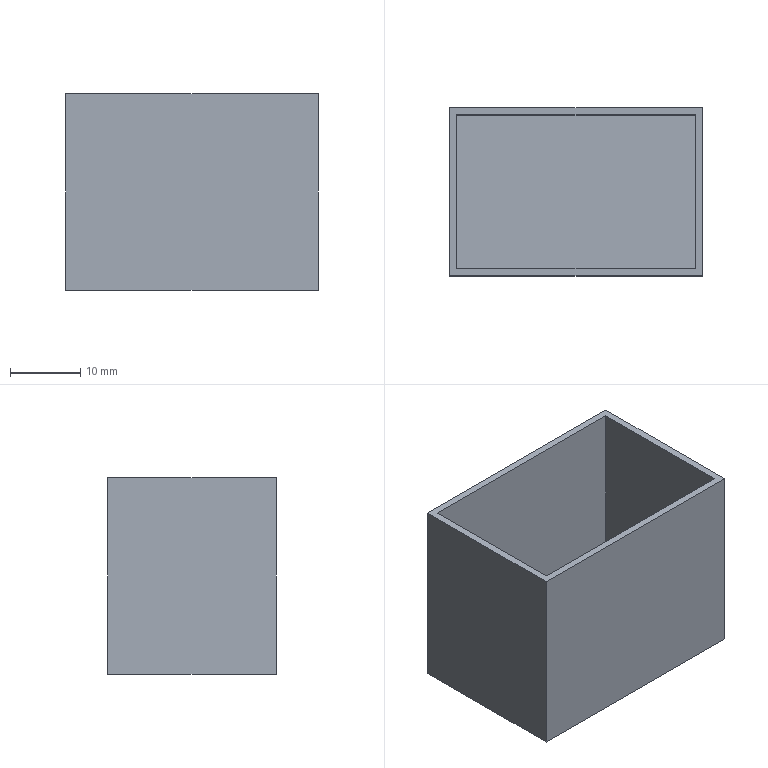Component | NX | MATERIAL_COLLECTION_BOX | 1 solid | 11 faces | box 36 x 24 x 28 mm | volume 3996 mm3 | plane 11
STEP:
#1=CARTESIAN_POINT('',(0.,0.,0.));
#2=DIRECTION('',(0.,0.,1.));
#3=DIRECTION('',(1.,0.,0.));
#4=AXIS2_PLACEMENT_3D('',#1,#2,#3);
#5=CARTESIAN_POINT('',(-110.,4.498,6.));
#6=VERTEX_POINT('',#5);
#7=CARTESIAN_POINT('',(-146.,4.498,6.));
#8=VERTEX_POINT('',#7);
#9=CARTESIAN_POINT('',(-128.,4.498,6.));
#10=DIRECTION('',(-1.,0.,0.));
#11=VECTOR('',#10,1.);
#12=LINE('',#9,#11);
#13=CARTESIAN_POINT('',(-128.,16.498,6.));
#14=DIRECTION('',(0.,0.,1.));
#15=DIRECTION('',(1.,0.,0.));
#16=AXIS2_PLACEMENT_3D('',#13,#14,#15);
#17=PLANE('',#16);
#18=CARTESIAN_POINT('',(0.,-12.));
#19=DIRECTION('',(-1.,0.));
#20=VECTOR('',#19,1.);
#21=LINE('',#18,#20);
#22=(GEOMETRIC_REPRESENTATION_CONTEXT(2)PARAMETRIC_REPRESENTATION_CONTEXT()REPRESENTATION_CONTEXT('',''));
#23=DEFINITIONAL_REPRESENTATION('',(#21),#22);
#24=PCURVE('',#17,#23);
#25=CARTESIAN_POINT('',(-128.,4.498,-22.));
#26=DIRECTION('',(0.,-1.,0.));
#27=DIRECTION('',(0.,0.,-1.));
#28=AXIS2_PLACEMENT_3D('',#25,#26,#27);
#29=PLANE('',#28);
#30=CARTESIAN_POINT('',(-28.,0.));
#31=DIRECTION('',(0.,-1.));
#32=VECTOR('',#31,1.);
#33=LINE('',#30,#32);
#34=(GEOMETRIC_REPRESENTATION_CONTEXT(2)PARAMETRIC_REPRESENTATION_CONTEXT()REPRESENTATION_CONTEXT('',''));
#35=DEFINITIONAL_REPRESENTATION('',(#33),#34);
#36=PCURVE('',#29,#35);
#37=SURFACE_CURVE('',#12,(#24,#36),.PCURVE_S1.);
#38=EDGE_CURVE('',#6,#8,#37,.T.);
#39=ORIENTED_EDGE('',*,*,#38,.F.);
#40=CARTESIAN_POINT('',(-110.,28.498,6.));
#41=VERTEX_POINT('',#40);
#42=CARTESIAN_POINT('',(-110.,16.498,6.));
#43=DIRECTION('',(0.,-1.,0.));
#44=VECTOR('',#43,1.);
#45=LINE('',#42,#44);
#46=CARTESIAN_POINT('',(18.,0.));
#47=DIRECTION('',(0.,-1.));
#48=VECTOR('',#47,1.);
#49=LINE('',#46,#48);
#50=(GEOMETRIC_REPRESENTATION_CONTEXT(2)PARAMETRIC_REPRESENTATION_CONTEXT()REPRESENTATION_CONTEXT('',''));
#51=DEFINITIONAL_REPRESENTATION('',(#49),#50);
#52=PCURVE('',#17,#51);
#53=CARTESIAN_POINT('',(-110.,16.498,-22.));
#54=DIRECTION('',(1.,0.,0.));
#55=DIRECTION('',(0.,0.,-1.));
#56=AXIS2_PLACEMENT_3D('',#53,#54,#55);
#57=PLANE('',#56);
#58=CARTESIAN_POINT('',(-28.,0.));
#59=DIRECTION('',(0.,-1.));
#60=VECTOR('',#59,1.);
#61=LINE('',#58,#60);
#62=(GEOMETRIC_REPRESENTATION_CONTEXT(2)PARAMETRIC_REPRESENTATION_CONTEXT()REPRESENTATION_CONTEXT('',''));
#63=DEFINITIONAL_REPRESENTATION('',(#61),#62);
#64=PCURVE('',#57,#63);
#65=SURFACE_CURVE('',#45,(#52,#64),.PCURVE_S1.);
#66=EDGE_CURVE('',#41,#6,#65,.T.);
#67=ORIENTED_EDGE('',*,*,#66,.F.);
#68=CARTESIAN_POINT('',(-146.,28.498,6.));
#69=VERTEX_POINT('',#68);
#70=CARTESIAN_POINT('',(-128.,28.498,6.));
#71=DIRECTION('',(1.,0.,0.));
#72=VECTOR('',#71,1.);
#73=LINE('',#70,#72);
#74=CARTESIAN_POINT('',(0.,12.));
#75=DIRECTION('',(1.,0.));
#76=VECTOR('',#75,1.);
#77=LINE('',#74,#76);
#78=(GEOMETRIC_REPRESENTATION_CONTEXT(2)PARAMETRIC_REPRESENTATION_CONTEXT()REPRESENTATION_CONTEXT('',''));
#79=DEFINITIONAL_REPRESENTATION('',(#77),#78);
#80=PCURVE('',#17,#79);
#81=CARTESIAN_POINT('',(-128.,28.498,-22.));
#82=DIRECTION('',(0.,1.,0.));
#83=DIRECTION('',(0.,0.,1.));
#84=AXIS2_PLACEMENT_3D('',#81,#82,#83);
#85=PLANE('',#84);
#86=CARTESIAN_POINT('',(28.,0.));
#87=DIRECTION('',(0.,1.));
#88=VECTOR('',#87,1.);
#89=LINE('',#86,#88);
#90=(GEOMETRIC_REPRESENTATION_CONTEXT(2)PARAMETRIC_REPRESENTATION_CONTEXT()REPRESENTATION_CONTEXT('',''));
#91=DEFINITIONAL_REPRESENTATION('',(#89),#90);
#92=PCURVE('',#85,#91);
#93=SURFACE_CURVE('',#73,(#80,#92),.PCURVE_S1.);
#94=EDGE_CURVE('',#69,#41,#93,.T.);
#95=ORIENTED_EDGE('',*,*,#94,.F.);
#96=CARTESIAN_POINT('',(-146.,16.498,6.));
#97=DIRECTION('',(0.,1.,0.));
#98=VECTOR('',#97,1.);
#99=LINE('',#96,#98);
#100=CARTESIAN_POINT('',(-18.,0.));
#101=DIRECTION('',(0.,1.));
#102=VECTOR('',#101,1.);
#103=LINE('',#100,#102);
#104=(GEOMETRIC_REPRESENTATION_CONTEXT(2)PARAMETRIC_REPRESENTATION_CONTEXT()REPRESENTATION_CONTEXT('',''));
#105=DEFINITIONAL_REPRESENTATION('',(#103),#104);
#106=PCURVE('',#17,#105);
#107=CARTESIAN_POINT('',(-146.,16.498,-22.));
#108=DIRECTION('',(-1.,0.,0.));
#109=DIRECTION('',(0.,0.,1.));
#110=AXIS2_PLACEMENT_3D('',#107,#108,#109);
#111=PLANE('',#110);
#112=CARTESIAN_POINT('',(28.,0.));
#113=DIRECTION('',(0.,1.));
#114=VECTOR('',#113,1.);
#115=LINE('',#112,#114);
#116=(GEOMETRIC_REPRESENTATION_CONTEXT(2)PARAMETRIC_REPRESENTATION_CONTEXT()REPRESENTATION_CONTEXT('',''));
#117=DEFINITIONAL_REPRESENTATION('',(#115),#116);
#118=PCURVE('',#111,#117);
#119=SURFACE_CURVE('',#99,(#106,#118),.PCURVE_S1.);
#120=EDGE_CURVE('',#8,#69,#119,.T.);
#121=ORIENTED_EDGE('',*,*,#120,.F.);
#122=EDGE_LOOP('',(#39,#67,#95,#121));
#123=FACE_BOUND('',#122,.T.);
#124=CARTESIAN_POINT('',(-111.,27.498,6.));
#125=VERTEX_POINT('',#124);
#126=CARTESIAN_POINT('',(-111.,5.498,6.));
#127=VERTEX_POINT('',#126);
#128=CARTESIAN_POINT('',(-111.,16.498,6.));
#129=DIRECTION('',(0.,-1.,0.));
#130=VECTOR('',#129,1.);
#131=LINE('',#128,#130);
#132=CARTESIAN_POINT('',(17.,0.));
#133=DIRECTION('',(0.,-1.));
#134=VECTOR('',#133,1.);
#135=LINE('',#132,#134);
#136=(GEOMETRIC_REPRESENTATION_CONTEXT(2)PARAMETRIC_REPRESENTATION_CONTEXT()REPRESENTATION_CONTEXT('',''));
#137=DEFINITIONAL_REPRESENTATION('',(#135),#136);
#138=PCURVE('',#17,#137);
#139=CARTESIAN_POINT('',(-111.,16.498,-22.));
#140=DIRECTION('',(1.,0.,0.));
#141=DIRECTION('',(0.,0.,-1.));
#142=AXIS2_PLACEMENT_3D('',#139,#140,#141);
#143=PLANE('',#142);
#144=CARTESIAN_POINT('',(-28.,0.));
#145=DIRECTION('',(0.,-1.));
#146=VECTOR('',#145,1.);
#147=LINE('',#144,#146);
#148=(GEOMETRIC_REPRESENTATION_CONTEXT(2)PARAMETRIC_REPRESENTATION_CONTEXT()REPRESENTATION_CONTEXT('',''));
#149=DEFINITIONAL_REPRESENTATION('',(#147),#148);
#150=PCURVE('',#143,#149);
#151=SURFACE_CURVE('',#131,(#138,#150),.PCURVE_S1.);
#152=EDGE_CURVE('',#125,#127,#151,.T.);
#153=ORIENTED_EDGE('',*,*,#152,.T.);
#154=CARTESIAN_POINT('',(-145.,5.498,6.));
#155=VERTEX_POINT('',#154);
#156=CARTESIAN_POINT('',(-128.,5.498,6.));
#157=DIRECTION('',(-1.,0.,0.));
#158=VECTOR('',#157,1.);
#159=LINE('',#156,#158);
#160=CARTESIAN_POINT('',(0.,-11.));
#161=DIRECTION('',(-1.,0.));
#162=VECTOR('',#161,1.);
#163=LINE('',#160,#162);
#164=(GEOMETRIC_REPRESENTATION_CONTEXT(2)PARAMETRIC_REPRESENTATION_CONTEXT()REPRESENTATION_CONTEXT('',''));
#165=DEFINITIONAL_REPRESENTATION('',(#163),#164);
#166=PCURVE('',#17,#165);
#167=CARTESIAN_POINT('',(-128.,5.498,-22.));
#168=DIRECTION('',(0.,-1.,0.));
#169=DIRECTION('',(0.,0.,-1.));
#170=AXIS2_PLACEMENT_3D('',#167,#168,#169);
#171=PLANE('',#170);
#172=CARTESIAN_POINT('',(-28.,0.));
#173=DIRECTION('',(0.,-1.));
#174=VECTOR('',#173,1.);
#175=LINE('',#172,#174);
#176=(GEOMETRIC_REPRESENTATION_CONTEXT(2)PARAMETRIC_REPRESENTATION_CONTEXT()REPRESENTATION_CONTEXT('',''));
#177=DEFINITIONAL_REPRESENTATION('',(#175),#176);
#178=PCURVE('',#171,#177);
#179=SURFACE_CURVE('',#159,(#166,#178),.PCURVE_S1.);
#180=EDGE_CURVE('',#127,#155,#179,.T.);
#181=ORIENTED_EDGE('',*,*,#180,.T.);
#182=CARTESIAN_POINT('',(-145.,27.498,6.));
#183=VERTEX_POINT('',#182);
#184=CARTESIAN_POINT('',(-145.,16.498,6.));
#185=DIRECTION('',(0.,1.,0.));
#186=VECTOR('',#185,1.);
#187=LINE('',#184,#186);
#188=CARTESIAN_POINT('',(-17.,0.));
#189=DIRECTION('',(0.,1.));
#190=VECTOR('',#189,1.);
#191=LINE('',#188,#190);
#192=(GEOMETRIC_REPRESENTATION_CONTEXT(2)PARAMETRIC_REPRESENTATION_CONTEXT()REPRESENTATION_CONTEXT('',''));
#193=DEFINITIONAL_REPRESENTATION('',(#191),#192);
#194=PCURVE('',#17,#193);
#195=CARTESIAN_POINT('',(-145.,16.498,-22.));
#196=DIRECTION('',(-1.,0.,0.));
#197=DIRECTION('',(0.,0.,1.));
#198=AXIS2_PLACEMENT_3D('',#195,#196,#197);
#199=PLANE('',#198);
#200=CARTESIAN_POINT('',(28.,0.));
#201=DIRECTION('',(0.,1.));
#202=VECTOR('',#201,1.);
#203=LINE('',#200,#202);
#204=(GEOMETRIC_REPRESENTATION_CONTEXT(2)PARAMETRIC_REPRESENTATION_CONTEXT()REPRESENTATION_CONTEXT('',''));
#205=DEFINITIONAL_REPRESENTATION('',(#203),#204);
#206=PCURVE('',#199,#205);
#207=SURFACE_CURVE('',#187,(#194,#206),.PCURVE_S1.);
#208=EDGE_CURVE('',#155,#183,#207,.T.);
#209=ORIENTED_EDGE('',*,*,#208,.T.);
#210=CARTESIAN_POINT('',(-128.,27.498,6.));
#211=DIRECTION('',(1.,0.,0.));
#212=VECTOR('',#211,1.);
#213=LINE('',#210,#212);
#214=CARTESIAN_POINT('',(0.,11.));
#215=DIRECTION('',(1.,0.));
#216=VECTOR('',#215,1.);
#217=LINE('',#214,#216);
#218=(GEOMETRIC_REPRESENTATION_CONTEXT(2)PARAMETRIC_REPRESENTATION_CONTEXT()REPRESENTATION_CONTEXT('',''));
#219=DEFINITIONAL_REPRESENTATION('',(#217),#218);
#220=PCURVE('',#17,#219);
#221=CARTESIAN_POINT('',(-128.,27.498,-22.));
#222=DIRECTION('',(0.,1.,0.));
#223=DIRECTION('',(0.,0.,1.));
#224=AXIS2_PLACEMENT_3D('',#221,#222,#223);
#225=PLANE('',#224);
#226=CARTESIAN_POINT('',(28.,0.));
#227=DIRECTION('',(0.,1.));
#228=VECTOR('',#227,1.);
#229=LINE('',#226,#228);
#230=(GEOMETRIC_REPRESENTATION_CONTEXT(2)PARAMETRIC_REPRESENTATION_CONTEXT()REPRESENTATION_CONTEXT('',''));
#231=DEFINITIONAL_REPRESENTATION('',(#229),#230);
#232=PCURVE('',#225,#231);
#233=SURFACE_CURVE('',#213,(#220,#232),.PCURVE_S1.);
#234=EDGE_CURVE('',#183,#125,#233,.T.);
#235=ORIENTED_EDGE('',*,*,#234,.T.);
#236=EDGE_LOOP('',(#153,#181,#209,#235));
#237=FACE_BOUND('',#236,.T.);
#238=ADVANCED_FACE('',(#123,#237),#17,.T.);
#239=CARTESIAN_POINT('',(-110.,4.498,-22.));
#240=VERTEX_POINT('',#239);
#241=CARTESIAN_POINT('',(-110.,4.498,-22.));
#242=DIRECTION('',(0.,0.,1.));
#243=VECTOR('',#242,1.);
#244=LINE('',#241,#243);
#245=CARTESIAN_POINT('',(0.,18.));
#246=DIRECTION('',(-1.,0.));
#247=VECTOR('',#246,1.);
#248=LINE('',#245,#247);
#249=(GEOMETRIC_REPRESENTATION_CONTEXT(2)PARAMETRIC_REPRESENTATION_CONTEXT()REPRESENTATION_CONTEXT('',''));
#250=DEFINITIONAL_REPRESENTATION('',(#248),#249);
#251=PCURVE('',#29,#250);
#252=CARTESIAN_POINT('',(0.,-12.));
#253=DIRECTION('',(-1.,0.));
#254=VECTOR('',#253,1.);
#255=LINE('',#252,#254);
#256=(GEOMETRIC_REPRESENTATION_CONTEXT(2)PARAMETRIC_REPRESENTATION_CONTEXT()REPRESENTATION_CONTEXT('',''));
#257=DEFINITIONAL_REPRESENTATION('',(#255),#256);
#258=PCURVE('',#57,#257);
#259=SURFACE_CURVE('',#244,(#251,#258),.PCURVE_S1.);
#260=EDGE_CURVE('',#240,#6,#259,.T.);
#261=ORIENTED_EDGE('',*,*,#260,.T.);
#262=ORIENTED_EDGE('',*,*,#38,.T.);
#263=CARTESIAN_POINT('',(-146.,4.498,-22.));
#264=VERTEX_POINT('',#263);
#265=CARTESIAN_POINT('',(-146.,4.498,-22.));
#266=DIRECTION('',(0.,0.,1.));
#267=VECTOR('',#266,1.);
#268=LINE('',#265,#267);
#269=CARTESIAN_POINT('',(0.,-18.));
#270=DIRECTION('',(-1.,0.));
#271=VECTOR('',#270,1.);
#272=LINE('',#269,#271);
#273=(GEOMETRIC_REPRESENTATION_CONTEXT(2)PARAMETRIC_REPRESENTATION_CONTEXT()REPRESENTATION_CONTEXT('',''));
#274=DEFINITIONAL_REPRESENTATION('',(#272),#273);
#275=PCURVE('',#29,#274);
#276=CARTESIAN_POINT('',(0.,-12.));
#277=DIRECTION('',(1.,0.));
#278=VECTOR('',#277,1.);
#279=LINE('',#276,#278);
#280=(GEOMETRIC_REPRESENTATION_CONTEXT(2)PARAMETRIC_REPRESENTATION_CONTEXT()REPRESENTATION_CONTEXT('',''));
#281=DEFINITIONAL_REPRESENTATION('',(#279),#280);
#282=PCURVE('',#111,#281);
#283=SURFACE_CURVE('',#268,(#275,#282),.PCURVE_S1.);
#284=EDGE_CURVE('',#264,#8,#283,.T.);
#285=ORIENTED_EDGE('',*,*,#284,.F.);
#286=CARTESIAN_POINT('',(-128.,4.498,-22.));
#287=DIRECTION('',(1.,0.,0.));
#288=VECTOR('',#287,1.);
#289=LINE('',#286,#288);
#290=CARTESIAN_POINT('',(0.,0.));
#291=DIRECTION('',(0.,1.));
#292=VECTOR('',#291,1.);
#293=LINE('',#290,#292);
#294=(GEOMETRIC_REPRESENTATION_CONTEXT(2)PARAMETRIC_REPRESENTATION_CONTEXT()REPRESENTATION_CONTEXT('',''));
#295=DEFINITIONAL_REPRESENTATION('',(#293),#294);
#296=PCURVE('',#29,#295);
#297=CARTESIAN_POINT('',(-128.,16.498,-22.));
#298=DIRECTION('',(0.,0.,-1.));
#299=DIRECTION('',(-1.,0.,0.));
#300=AXIS2_PLACEMENT_3D('',#297,#298,#299);
#301=PLANE('',#300);
#302=CARTESIAN_POINT('',(0.,-12.));
#303=DIRECTION('',(-1.,0.));
#304=VECTOR('',#303,1.);
#305=LINE('',#302,#304);
#306=(GEOMETRIC_REPRESENTATION_CONTEXT(2)PARAMETRIC_REPRESENTATION_CONTEXT()REPRESENTATION_CONTEXT('',''));
#307=DEFINITIONAL_REPRESENTATION('',(#305),#306);
#308=PCURVE('',#301,#307);
#309=SURFACE_CURVE('',#289,(#296,#308),.PCURVE_S1.);
#310=EDGE_CURVE('',#264,#240,#309,.T.);
#311=ORIENTED_EDGE('',*,*,#310,.T.);
#312=EDGE_LOOP('',(#261,#262,#285,#311));
#313=FACE_BOUND('',#312,.T.);
#314=ADVANCED_FACE('',(#313),#29,.T.);
#315=ORIENTED_EDGE('',*,*,#284,.T.);
#316=ORIENTED_EDGE('',*,*,#120,.T.);
#317=CARTESIAN_POINT('',(-146.,28.498,-22.));
#318=VERTEX_POINT('',#317);
#319=CARTESIAN_POINT('',(-146.,28.498,-22.));
#320=DIRECTION('',(0.,0.,1.));
#321=VECTOR('',#320,1.);
#322=LINE('',#319,#321);
#323=CARTESIAN_POINT('',(0.,12.));
#324=DIRECTION('',(1.,0.));
#325=VECTOR('',#324,1.);
#326=LINE('',#323,#325);
#327=(GEOMETRIC_REPRESENTATION_CONTEXT(2)PARAMETRIC_REPRESENTATION_CONTEXT()REPRESENTATION_CONTEXT('',''));
#328=DEFINITIONAL_REPRESENTATION('',(#326),#327);
#329=PCURVE('',#111,#328);
#330=CARTESIAN_POINT('',(0.,-18.));
#331=DIRECTION('',(1.,0.));
#332=VECTOR('',#331,1.);
#333=LINE('',#330,#332);
#334=(GEOMETRIC_REPRESENTATION_CONTEXT(2)PARAMETRIC_REPRESENTATION_CONTEXT()REPRESENTATION_CONTEXT('',''));
#335=DEFINITIONAL_REPRESENTATION('',(#333),#334);
#336=PCURVE('',#85,#335);
#337=SURFACE_CURVE('',#322,(#329,#336),.PCURVE_S1.);
#338=EDGE_CURVE('',#318,#69,#337,.T.);
#339=ORIENTED_EDGE('',*,*,#338,.F.);
#340=CARTESIAN_POINT('',(-146.,16.498,-22.));
#341=DIRECTION('',(0.,-1.,0.));
#342=VECTOR('',#341,1.);
#343=LINE('',#340,#342);
#344=CARTESIAN_POINT('',(0.,0.));
#345=DIRECTION('',(0.,-1.));
#346=VECTOR('',#345,1.);
#347=LINE('',#344,#346);
#348=(GEOMETRIC_REPRESENTATION_CONTEXT(2)PARAMETRIC_REPRESENTATION_CONTEXT()REPRESENTATION_CONTEXT('',''));
#349=DEFINITIONAL_REPRESENTATION('',(#347),#348);
#350=PCURVE('',#111,#349);
#351=CARTESIAN_POINT('',(18.,0.));
#352=DIRECTION('',(0.,-1.));
#353=VECTOR('',#352,1.);
#354=LINE('',#351,#353);
#355=(GEOMETRIC_REPRESENTATION_CONTEXT(2)PARAMETRIC_REPRESENTATION_CONTEXT()REPRESENTATION_CONTEXT('',''));
#356=DEFINITIONAL_REPRESENTATION('',(#354),#355);
#357=PCURVE('',#301,#356);
#358=SURFACE_CURVE('',#343,(#350,#357),.PCURVE_S1.);
#359=EDGE_CURVE('',#318,#264,#358,.T.);
#360=ORIENTED_EDGE('',*,*,#359,.T.);
#361=EDGE_LOOP('',(#315,#316,#339,#360));
#362=FACE_BOUND('',#361,.T.);
#363=ADVANCED_FACE('',(#362),#111,.T.);
#364=ORIENTED_EDGE('',*,*,#338,.T.);
#365=ORIENTED_EDGE('',*,*,#94,.T.);
#366=CARTESIAN_POINT('',(-110.,28.498,-22.));
#367=VERTEX_POINT('',#366);
#368=CARTESIAN_POINT('',(-110.,28.498,-22.));
#369=DIRECTION('',(0.,0.,1.));
#370=VECTOR('',#369,1.);
#371=LINE('',#368,#370);
#372=CARTESIAN_POINT('',(0.,18.));
#373=DIRECTION('',(1.,0.));
#374=VECTOR('',#373,1.);
#375=LINE('',#372,#374);
#376=(GEOMETRIC_REPRESENTATION_CONTEXT(2)PARAMETRIC_REPRESENTATION_CONTEXT()REPRESENTATION_CONTEXT('',''));
#377=DEFINITIONAL_REPRESENTATION('',(#375),#376);
#378=PCURVE('',#85,#377);
#379=CARTESIAN_POINT('',(0.,12.));
#380=DIRECTION('',(-1.,0.));
#381=VECTOR('',#380,1.);
#382=LINE('',#379,#381);
#383=(GEOMETRIC_REPRESENTATION_CONTEXT(2)PARAMETRIC_REPRESENTATION_CONTEXT()REPRESENTATION_CONTEXT('',''));
#384=DEFINITIONAL_REPRESENTATION('',(#382),#383);
#385=PCURVE('',#57,#384);
#386=SURFACE_CURVE('',#371,(#378,#385),.PCURVE_S1.);
#387=EDGE_CURVE('',#367,#41,#386,.T.);
#388=ORIENTED_EDGE('',*,*,#387,.F.);
#389=CARTESIAN_POINT('',(-128.,28.498,-22.));
#390=DIRECTION('',(-1.,0.,0.));
#391=VECTOR('',#390,1.);
#392=LINE('',#389,#391);
#393=CARTESIAN_POINT('',(0.,0.));
#394=DIRECTION('',(0.,-1.));
#395=VECTOR('',#394,1.);
#396=LINE('',#393,#395);
#397=(GEOMETRIC_REPRESENTATION_CONTEXT(2)PARAMETRIC_REPRESENTATION_CONTEXT()REPRESENTATION_CONTEXT('',''));
#398=DEFINITIONAL_REPRESENTATION('',(#396),#397);
#399=PCURVE('',#85,#398);
#400=CARTESIAN_POINT('',(0.,12.));
#401=DIRECTION('',(1.,0.));
#402=VECTOR('',#401,1.);
#403=LINE('',#400,#402);
#404=(GEOMETRIC_REPRESENTATION_CONTEXT(2)PARAMETRIC_REPRESENTATION_CONTEXT()REPRESENTATION_CONTEXT('',''));
#405=DEFINITIONAL_REPRESENTATION('',(#403),#404);
#406=PCURVE('',#301,#405);
#407=SURFACE_CURVE('',#392,(#399,#406),.PCURVE_S1.);
#408=EDGE_CURVE('',#367,#318,#407,.T.);
#409=ORIENTED_EDGE('',*,*,#408,.T.);
#410=EDGE_LOOP('',(#364,#365,#388,#409));
#411=FACE_BOUND('',#410,.T.);
#412=ADVANCED_FACE('',(#411),#85,.T.);
#413=CARTESIAN_POINT('',(-110.,16.498,-22.));
#414=DIRECTION('',(0.,1.,0.));
#415=VECTOR('',#414,1.);
#416=LINE('',#413,#415);
#417=CARTESIAN_POINT('',(-18.,0.));
#418=DIRECTION('',(0.,1.));
#419=VECTOR('',#418,1.);
#420=LINE('',#417,#419);
#421=(GEOMETRIC_REPRESENTATION_CONTEXT(2)PARAMETRIC_REPRESENTATION_CONTEXT()REPRESENTATION_CONTEXT('',''));
#422=DEFINITIONAL_REPRESENTATION('',(#420),#421);
#423=PCURVE('',#301,#422);
#424=CARTESIAN_POINT('',(0.,0.));
#425=DIRECTION('',(0.,1.));
#426=VECTOR('',#425,1.);
#427=LINE('',#424,#426);
#428=(GEOMETRIC_REPRESENTATION_CONTEXT(2)PARAMETRIC_REPRESENTATION_CONTEXT()REPRESENTATION_CONTEXT('',''));
#429=DEFINITIONAL_REPRESENTATION('',(#427),#428);
#430=PCURVE('',#57,#429);
#431=SURFACE_CURVE('',#416,(#423,#430),.PCURVE_S1.);
#432=EDGE_CURVE('',#240,#367,#431,.T.);
#433=ORIENTED_EDGE('',*,*,#432,.F.);
#434=ORIENTED_EDGE('',*,*,#310,.F.);
#435=ORIENTED_EDGE('',*,*,#359,.F.);
#436=ORIENTED_EDGE('',*,*,#408,.F.);
#437=EDGE_LOOP('',(#433,#434,#435,#436));
#438=FACE_BOUND('',#437,.T.);
#439=ADVANCED_FACE('',(#438),#301,.T.);
#440=ORIENTED_EDGE('',*,*,#432,.T.);
#441=ORIENTED_EDGE('',*,*,#387,.T.);
#442=ORIENTED_EDGE('',*,*,#66,.T.);
#443=ORIENTED_EDGE('',*,*,#260,.F.);
#444=EDGE_LOOP('',(#440,#441,#442,#443));
#445=FACE_BOUND('',#444,.T.);
#446=ADVANCED_FACE('',(#445),#57,.T.);
#447=CARTESIAN_POINT('',(-111.,5.498,-21.));
#448=VERTEX_POINT('',#447);
#449=CARTESIAN_POINT('',(-111.,5.498,-22.));
#450=DIRECTION('',(0.,0.,1.));
#451=VECTOR('',#450,1.);
#452=LINE('',#449,#451);
#453=CARTESIAN_POINT('',(0.,17.));
#454=DIRECTION('',(-1.,0.));
#455=VECTOR('',#454,1.);
#456=LINE('',#453,#455);
#457=(GEOMETRIC_REPRESENTATION_CONTEXT(2)PARAMETRIC_REPRESENTATION_CONTEXT()REPRESENTATION_CONTEXT('',''));
#458=DEFINITIONAL_REPRESENTATION('',(#456),#457);
#459=PCURVE('',#171,#458);
#460=CARTESIAN_POINT('',(0.,-11.));
#461=DIRECTION('',(-1.,0.));
#462=VECTOR('',#461,1.);
#463=LINE('',#460,#462);
#464=(GEOMETRIC_REPRESENTATION_CONTEXT(2)PARAMETRIC_REPRESENTATION_CONTEXT()REPRESENTATION_CONTEXT('',''));
#465=DEFINITIONAL_REPRESENTATION('',(#463),#464);
#466=PCURVE('',#143,#465);
#467=SURFACE_CURVE('',#452,(#459,#466),.PCURVE_S1.);
#468=EDGE_CURVE('',#448,#127,#467,.T.);
#469=ORIENTED_EDGE('',*,*,#468,.F.);
#470=CARTESIAN_POINT('',(-145.,5.498,-21.));
#471=VERTEX_POINT('',#470);
#472=CARTESIAN_POINT('',(-128.,5.498,-21.));
#473=DIRECTION('',(1.,0.,0.));
#474=VECTOR('',#473,1.);
#475=LINE('',#472,#474);
#476=CARTESIAN_POINT('',(-1.,0.));
#477=DIRECTION('',(0.,1.));
#478=VECTOR('',#477,1.);
#479=LINE('',#476,#478);
#480=(GEOMETRIC_REPRESENTATION_CONTEXT(2)PARAMETRIC_REPRESENTATION_CONTEXT()REPRESENTATION_CONTEXT('',''));
#481=DEFINITIONAL_REPRESENTATION('',(#479),#480);
#482=PCURVE('',#171,#481);
#483=CARTESIAN_POINT('',(-128.,16.498,-21.));
#484=DIRECTION('',(0.,0.,-1.));
#485=DIRECTION('',(-1.,0.,0.));
#486=AXIS2_PLACEMENT_3D('',#483,#484,#485);
#487=PLANE('',#486);
#488=CARTESIAN_POINT('',(0.,-11.));
#489=DIRECTION('',(-1.,0.));
#490=VECTOR('',#489,1.);
#491=LINE('',#488,#490);
#492=(GEOMETRIC_REPRESENTATION_CONTEXT(2)PARAMETRIC_REPRESENTATION_CONTEXT()REPRESENTATION_CONTEXT('',''));
#493=DEFINITIONAL_REPRESENTATION('',(#491),#492);
#494=PCURVE('',#487,#493);
#495=SURFACE_CURVE('',#475,(#482,#494),.PCURVE_S1.);
#496=EDGE_CURVE('',#471,#448,#495,.T.);
#497=ORIENTED_EDGE('',*,*,#496,.F.);
#498=CARTESIAN_POINT('',(-145.,5.498,-22.));
#499=DIRECTION('',(0.,0.,1.));
#500=VECTOR('',#499,1.);
#501=LINE('',#498,#500);
#502=CARTESIAN_POINT('',(0.,-17.));
#503=DIRECTION('',(-1.,0.));
#504=VECTOR('',#503,1.);
#505=LINE('',#502,#504);
#506=(GEOMETRIC_REPRESENTATION_CONTEXT(2)PARAMETRIC_REPRESENTATION_CONTEXT()REPRESENTATION_CONTEXT('',''));
#507=DEFINITIONAL_REPRESENTATION('',(#505),#506);
#508=PCURVE('',#171,#507);
#509=CARTESIAN_POINT('',(0.,-11.));
#510=DIRECTION('',(1.,0.));
#511=VECTOR('',#510,1.);
#512=LINE('',#509,#511);
#513=(GEOMETRIC_REPRESENTATION_CONTEXT(2)PARAMETRIC_REPRESENTATION_CONTEXT()REPRESENTATION_CONTEXT('',''));
#514=DEFINITIONAL_REPRESENTATION('',(#512),#513);
#515=PCURVE('',#199,#514);
#516=SURFACE_CURVE('',#501,(#508,#515),.PCURVE_S1.);
#517=EDGE_CURVE('',#471,#155,#516,.T.);
#518=ORIENTED_EDGE('',*,*,#517,.T.);
#519=ORIENTED_EDGE('',*,*,#180,.F.);
#520=EDGE_LOOP('',(#469,#497,#518,#519));
#521=FACE_BOUND('',#520,.T.);
#522=ADVANCED_FACE('',(#521),#171,.F.);
#523=ORIENTED_EDGE('',*,*,#517,.F.);
#524=CARTESIAN_POINT('',(-145.,27.498,-21.));
#525=VERTEX_POINT('',#524);
#526=CARTESIAN_POINT('',(-145.,16.498,-21.));
#527=DIRECTION('',(0.,-1.,0.));
#528=VECTOR('',#527,1.);
#529=LINE('',#526,#528);
#530=CARTESIAN_POINT('',(1.,0.));
#531=DIRECTION('',(0.,-1.));
#532=VECTOR('',#531,1.);
#533=LINE('',#530,#532);
#534=(GEOMETRIC_REPRESENTATION_CONTEXT(2)PARAMETRIC_REPRESENTATION_CONTEXT()REPRESENTATION_CONTEXT('',''));
#535=DEFINITIONAL_REPRESENTATION('',(#533),#534);
#536=PCURVE('',#199,#535);
#537=CARTESIAN_POINT('',(17.,0.));
#538=DIRECTION('',(0.,-1.));
#539=VECTOR('',#538,1.);
#540=LINE('',#537,#539);
#541=(GEOMETRIC_REPRESENTATION_CONTEXT(2)PARAMETRIC_REPRESENTATION_CONTEXT()REPRESENTATION_CONTEXT('',''));
#542=DEFINITIONAL_REPRESENTATION('',(#540),#541);
#543=PCURVE('',#487,#542);
#544=SURFACE_CURVE('',#529,(#536,#543),.PCURVE_S1.);
#545=EDGE_CURVE('',#525,#471,#544,.T.);
#546=ORIENTED_EDGE('',*,*,#545,.F.);
#547=CARTESIAN_POINT('',(-145.,27.498,-22.));
#548=DIRECTION('',(0.,0.,1.));
#549=VECTOR('',#548,1.);
#550=LINE('',#547,#549);
#551=CARTESIAN_POINT('',(0.,11.));
#552=DIRECTION('',(1.,0.));
#553=VECTOR('',#552,1.);
#554=LINE('',#551,#553);
#555=(GEOMETRIC_REPRESENTATION_CONTEXT(2)PARAMETRIC_REPRESENTATION_CONTEXT()REPRESENTATION_CONTEXT('',''));
#556=DEFINITIONAL_REPRESENTATION('',(#554),#555);
#557=PCURVE('',#199,#556);
#558=CARTESIAN_POINT('',(0.,-17.));
#559=DIRECTION('',(1.,0.));
#560=VECTOR('',#559,1.);
#561=LINE('',#558,#560);
#562=(GEOMETRIC_REPRESENTATION_CONTEXT(2)PARAMETRIC_REPRESENTATION_CONTEXT()REPRESENTATION_CONTEXT('',''));
#563=DEFINITIONAL_REPRESENTATION('',(#561),#562);
#564=PCURVE('',#225,#563);
#565=SURFACE_CURVE('',#550,(#557,#564),.PCURVE_S1.);
#566=EDGE_CURVE('',#525,#183,#565,.T.);
#567=ORIENTED_EDGE('',*,*,#566,.T.);
#568=ORIENTED_EDGE('',*,*,#208,.F.);
#569=EDGE_LOOP('',(#523,#546,#567,#568));
#570=FACE_BOUND('',#569,.T.);
#571=ADVANCED_FACE('',(#570),#199,.F.);
#572=ORIENTED_EDGE('',*,*,#566,.F.);
#573=CARTESIAN_POINT('',(-111.,27.498,-21.));
#574=VERTEX_POINT('',#573);
#575=CARTESIAN_POINT('',(-128.,27.498,-21.));
#576=DIRECTION('',(-1.,0.,0.));
#577=VECTOR('',#576,1.);
#578=LINE('',#575,#577);
#579=CARTESIAN_POINT('',(1.,0.));
#580=DIRECTION('',(0.,-1.));
#581=VECTOR('',#580,1.);
#582=LINE('',#579,#581);
#583=(GEOMETRIC_REPRESENTATION_CONTEXT(2)PARAMETRIC_REPRESENTATION_CONTEXT()REPRESENTATION_CONTEXT('',''));
#584=DEFINITIONAL_REPRESENTATION('',(#582),#583);
#585=PCURVE('',#225,#584);
#586=CARTESIAN_POINT('',(0.,11.));
#587=DIRECTION('',(1.,0.));
#588=VECTOR('',#587,1.);
#589=LINE('',#586,#588);
#590=(GEOMETRIC_REPRESENTATION_CONTEXT(2)PARAMETRIC_REPRESENTATION_CONTEXT()REPRESENTATION_CONTEXT('',''));
#591=DEFINITIONAL_REPRESENTATION('',(#589),#590);
#592=PCURVE('',#487,#591);
#593=SURFACE_CURVE('',#578,(#585,#592),.PCURVE_S1.);
#594=EDGE_CURVE('',#574,#525,#593,.T.);
#595=ORIENTED_EDGE('',*,*,#594,.F.);
#596=CARTESIAN_POINT('',(-111.,27.498,-22.));
#597=DIRECTION('',(0.,0.,1.));
#598=VECTOR('',#597,1.);
#599=LINE('',#596,#598);
#600=CARTESIAN_POINT('',(0.,17.));
#601=DIRECTION('',(1.,0.));
#602=VECTOR('',#601,1.);
#603=LINE('',#600,#602);
#604=(GEOMETRIC_REPRESENTATION_CONTEXT(2)PARAMETRIC_REPRESENTATION_CONTEXT()REPRESENTATION_CONTEXT('',''));
#605=DEFINITIONAL_REPRESENTATION('',(#603),#604);
#606=PCURVE('',#225,#605);
#607=CARTESIAN_POINT('',(0.,11.));
#608=DIRECTION('',(-1.,0.));
#609=VECTOR('',#608,1.);
#610=LINE('',#607,#609);
#611=(GEOMETRIC_REPRESENTATION_CONTEXT(2)PARAMETRIC_REPRESENTATION_CONTEXT()REPRESENTATION_CONTEXT('',''));
#612=DEFINITIONAL_REPRESENTATION('',(#610),#611);
#613=PCURVE('',#143,#612);
#614=SURFACE_CURVE('',#599,(#606,#613),.PCURVE_S1.);
#615=EDGE_CURVE('',#574,#125,#614,.T.);
#616=ORIENTED_EDGE('',*,*,#615,.T.);
#617=ORIENTED_EDGE('',*,*,#234,.F.);
#618=EDGE_LOOP('',(#572,#595,#616,#617));
#619=FACE_BOUND('',#618,.T.);
#620=ADVANCED_FACE('',(#619),#225,.F.);
#621=CARTESIAN_POINT('',(-111.,16.498,-21.));
#622=DIRECTION('',(0.,1.,0.));
#623=VECTOR('',#622,1.);
#624=LINE('',#621,#623);
#625=CARTESIAN_POINT('',(-17.,0.));
#626=DIRECTION('',(0.,1.));
#627=VECTOR('',#626,1.);
#628=LINE('',#625,#627);
#629=(GEOMETRIC_REPRESENTATION_CONTEXT(2)PARAMETRIC_REPRESENTATION_CONTEXT()REPRESENTATION_CONTEXT('',''));
#630=DEFINITIONAL_REPRESENTATION('',(#628),#629);
#631=PCURVE('',#487,#630);
#632=CARTESIAN_POINT('',(-1.,0.));
#633=DIRECTION('',(0.,1.));
#634=VECTOR('',#633,1.);
#635=LINE('',#632,#634);
#636=(GEOMETRIC_REPRESENTATION_CONTEXT(2)PARAMETRIC_REPRESENTATION_CONTEXT()REPRESENTATION_CONTEXT('',''));
#637=DEFINITIONAL_REPRESENTATION('',(#635),#636);
#638=PCURVE('',#143,#637);
#639=SURFACE_CURVE('',#624,(#631,#638),.PCURVE_S1.);
#640=EDGE_CURVE('',#448,#574,#639,.T.);
#641=ORIENTED_EDGE('',*,*,#640,.T.);
#642=ORIENTED_EDGE('',*,*,#594,.T.);
#643=ORIENTED_EDGE('',*,*,#545,.T.);
#644=ORIENTED_EDGE('',*,*,#496,.T.);
#645=EDGE_LOOP('',(#641,#642,#643,#644));
#646=FACE_BOUND('',#645,.T.);
#647=ADVANCED_FACE('',(#646),#487,.F.);
#648=ORIENTED_EDGE('',*,*,#640,.F.);
#649=ORIENTED_EDGE('',*,*,#468,.T.);
#650=ORIENTED_EDGE('',*,*,#152,.F.);
#651=ORIENTED_EDGE('',*,*,#615,.F.);
#652=EDGE_LOOP('',(#648,#649,#650,#651));
#653=FACE_BOUND('',#652,.T.);
#654=ADVANCED_FACE('',(#653),#143,.F.);
#655=CLOSED_SHELL('',(#238,#314,#363,#412,#439,#446,#522,#571,#620,#647,#654));
#656=MANIFOLD_SOLID_BREP('',#655);
#657=(LENGTH_UNIT()NAMED_UNIT(*)SI_UNIT(.MILLI.,.METRE.));
#658=UNCERTAINTY_MEASURE_WITH_UNIT(LENGTH_MEASURE(0.0000001),#657,'','');
#659=(NAMED_UNIT(*)PLANE_ANGLE_UNIT()SI_UNIT($,.RADIAN.));
#660=(NAMED_UNIT(*)SI_UNIT($,.STERADIAN.)SOLID_ANGLE_UNIT());
#661=(GEOMETRIC_REPRESENTATION_CONTEXT(3)GLOBAL_UNCERTAINTY_ASSIGNED_CONTEXT((#658))GLOBAL_UNIT_ASSIGNED_CONTEXT((#657,#659,#660))REPRESENTATION_CONTEXT('',''));
#662=ADVANCED_BREP_SHAPE_REPRESENTATION('',(#4,#656),#661);